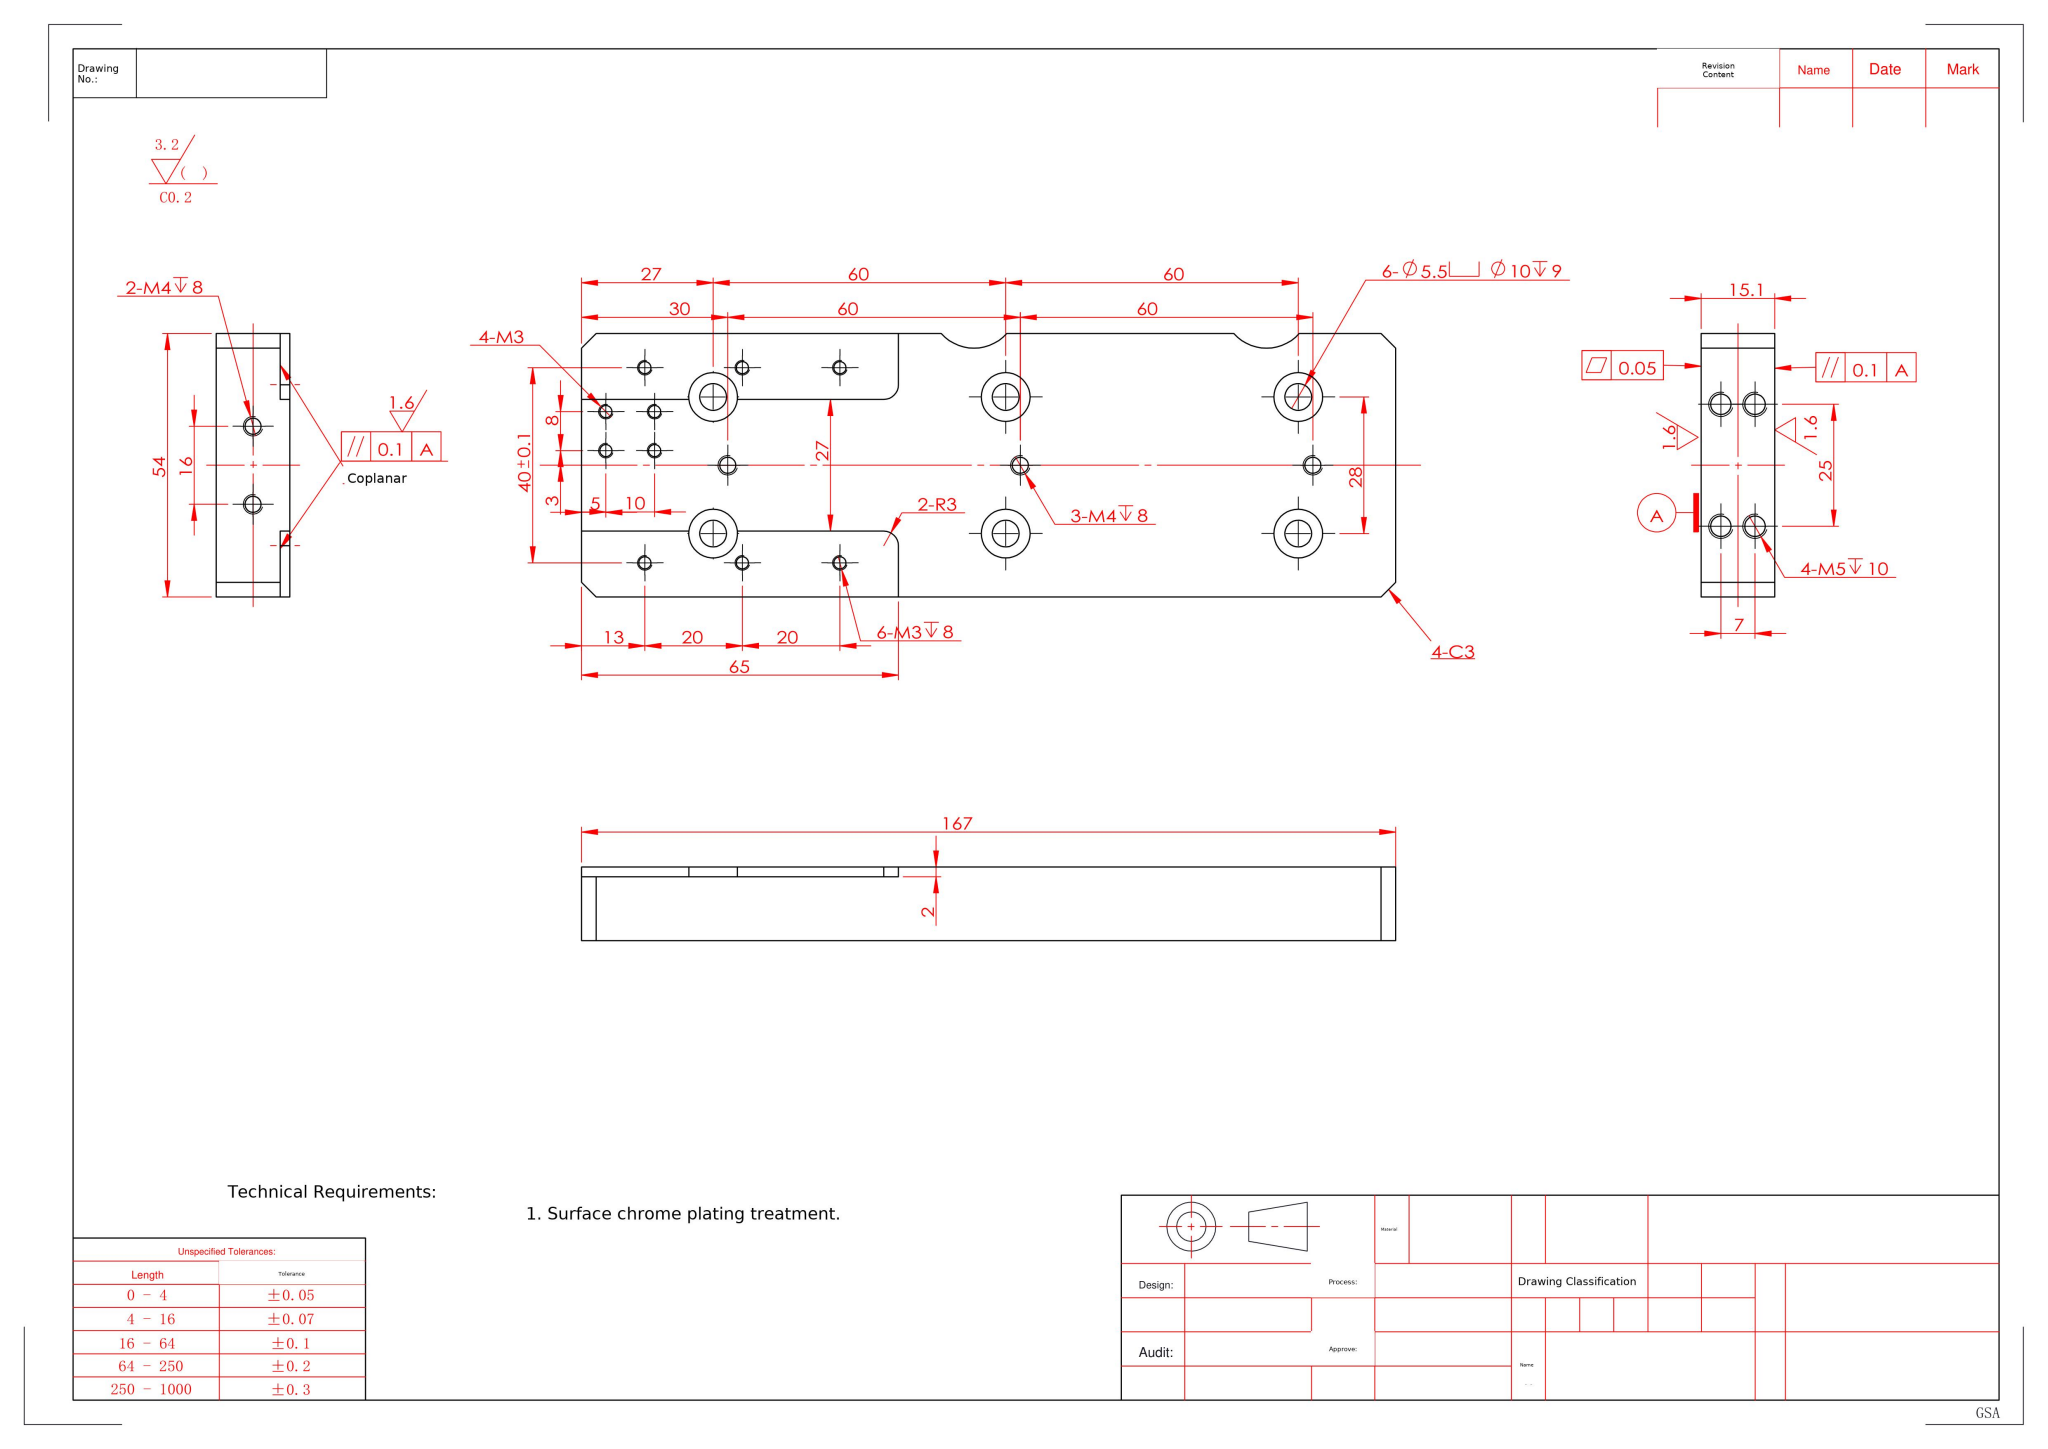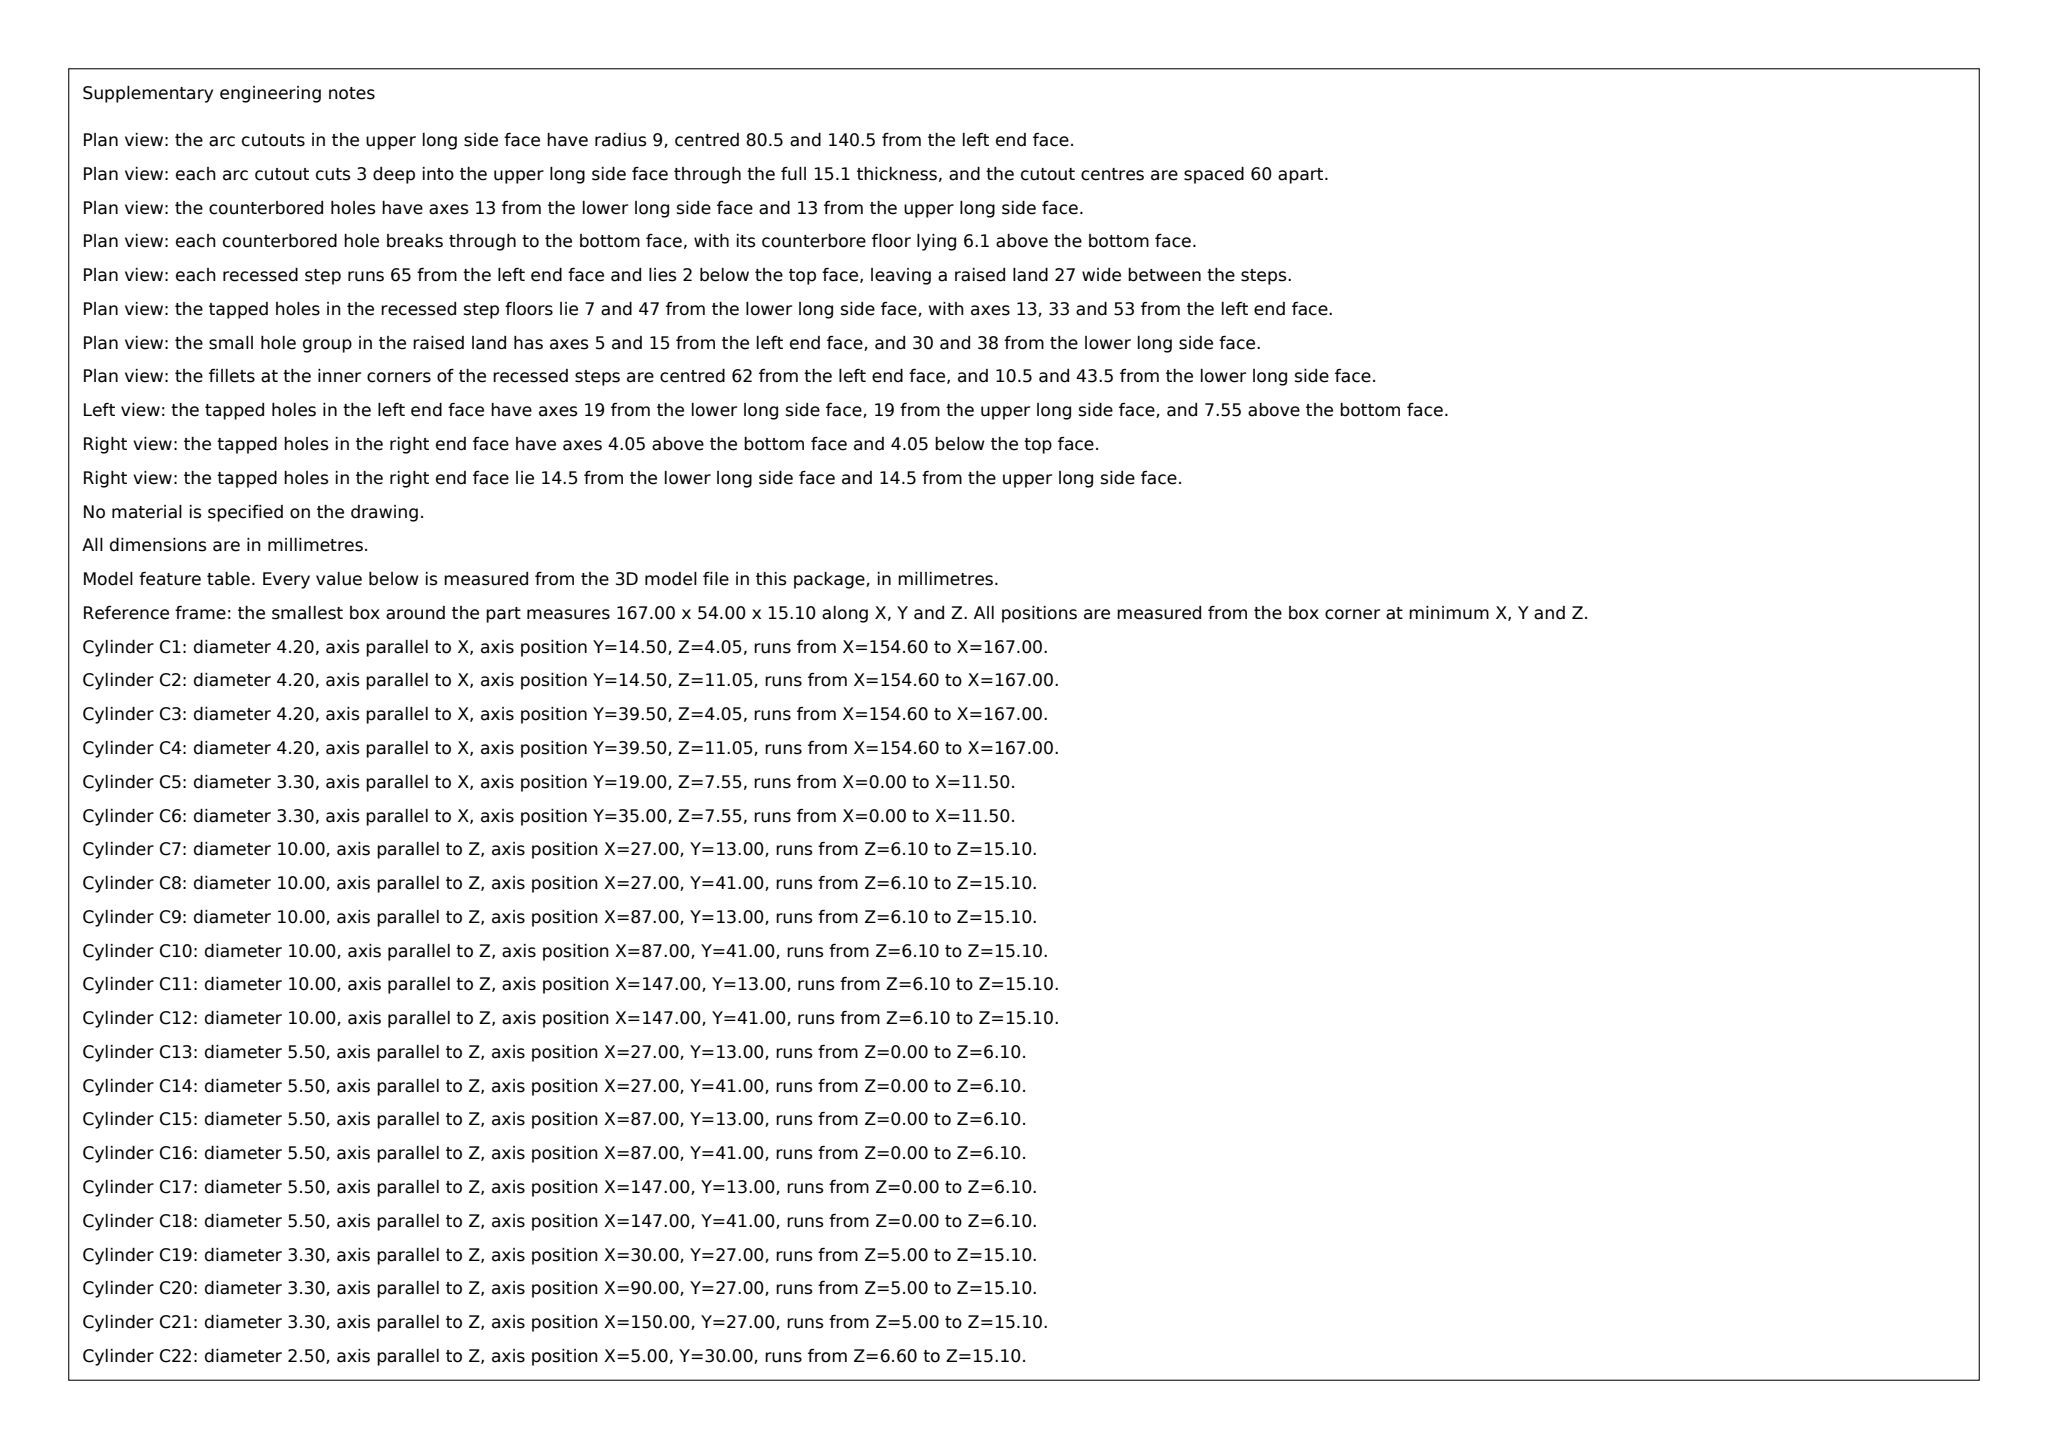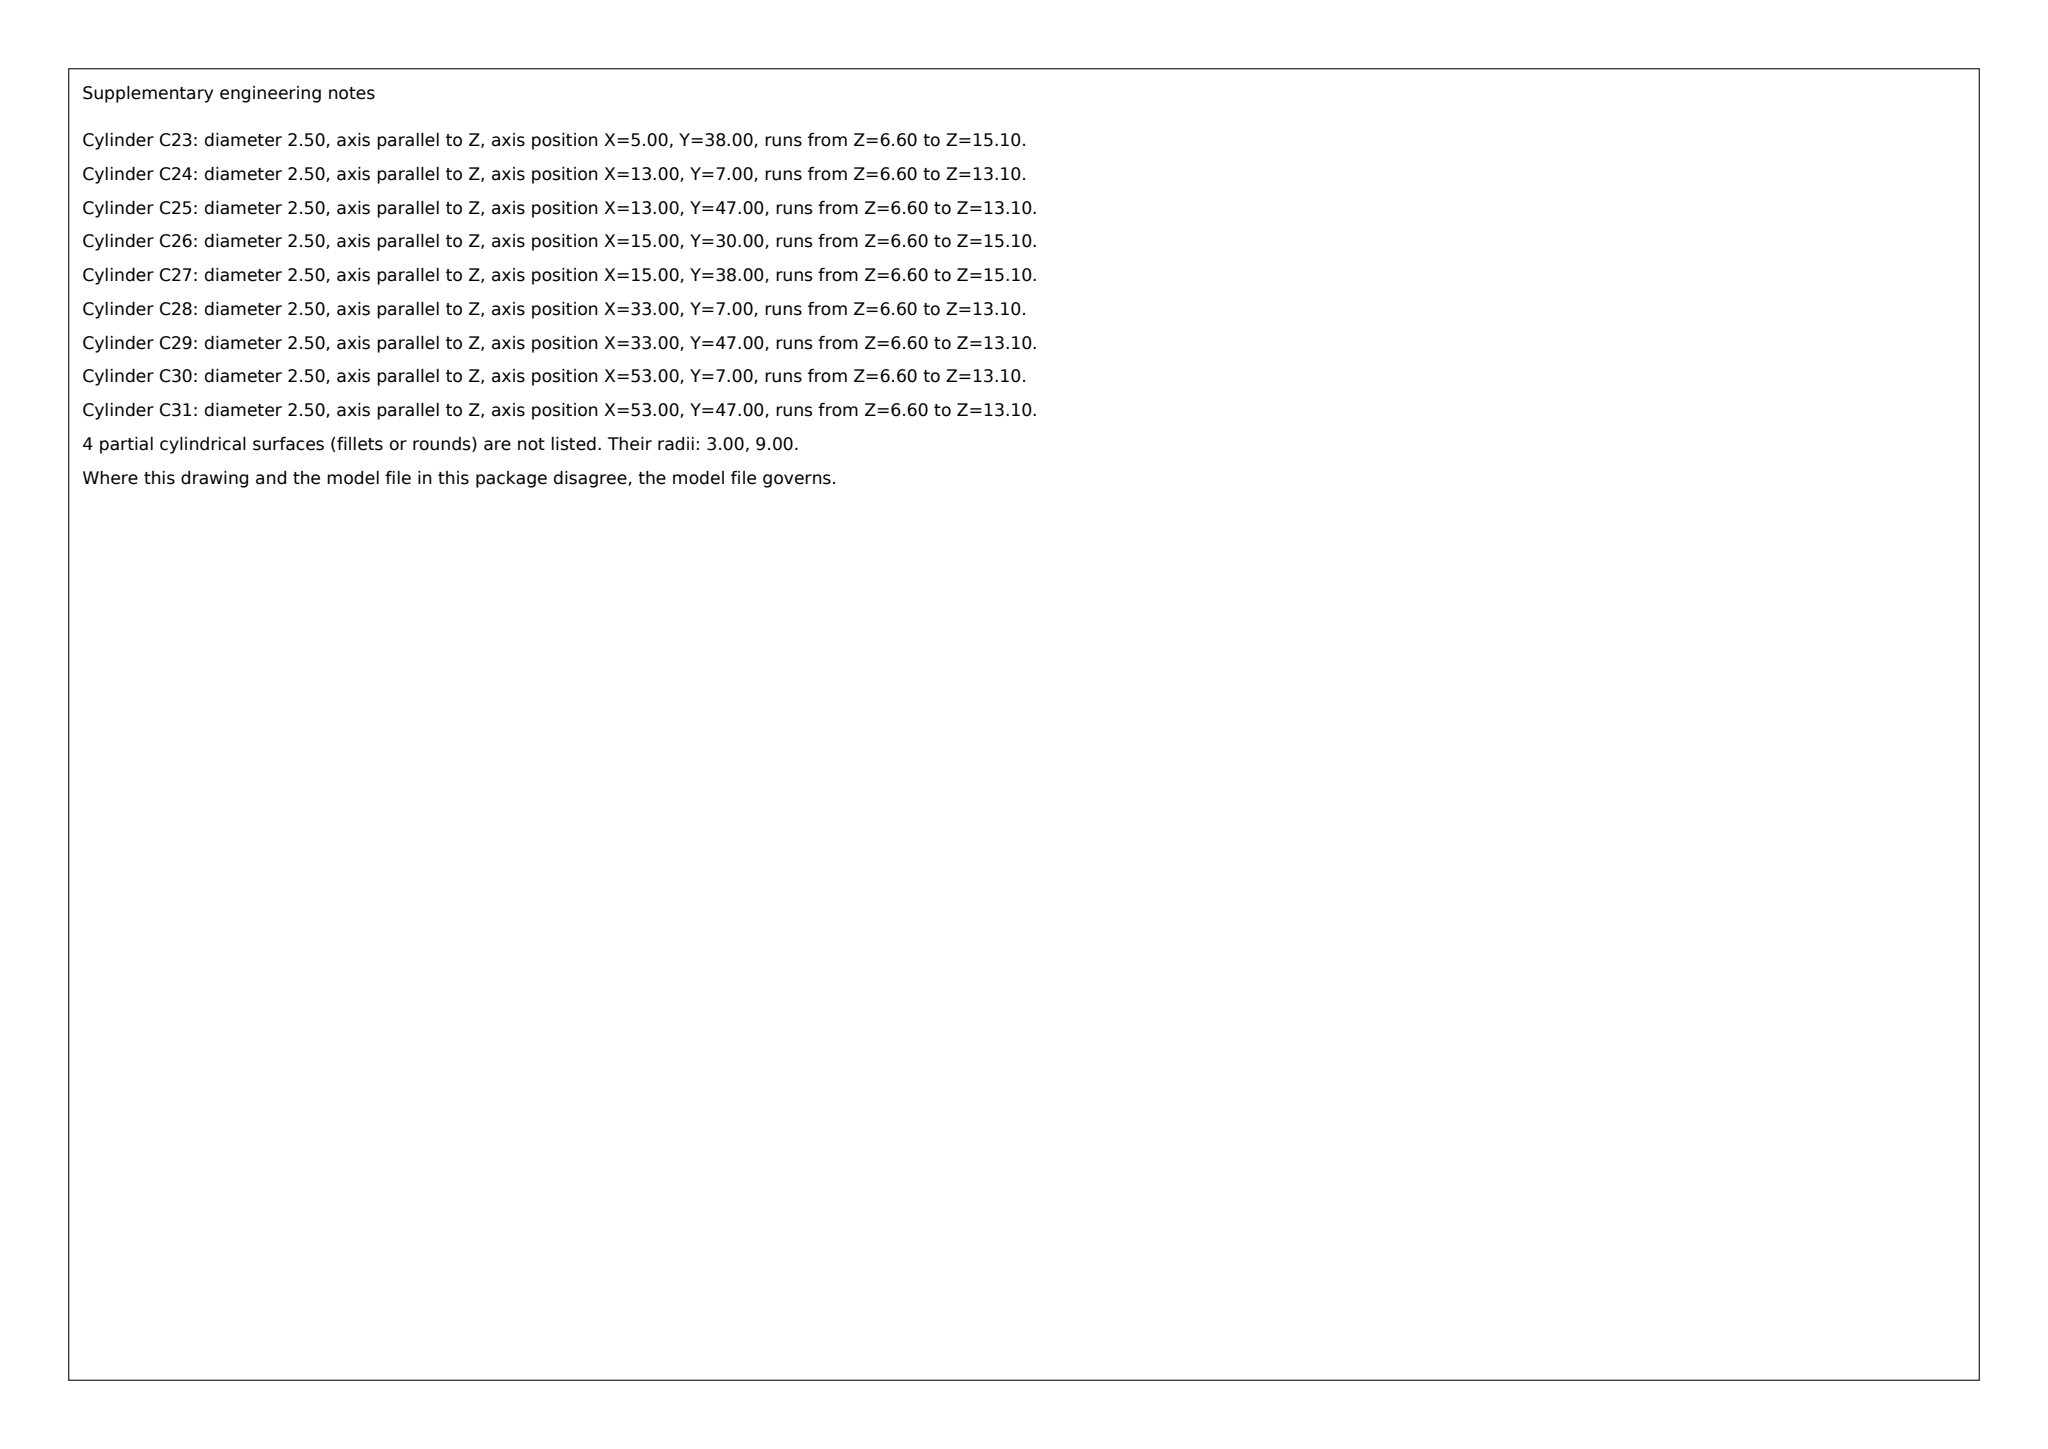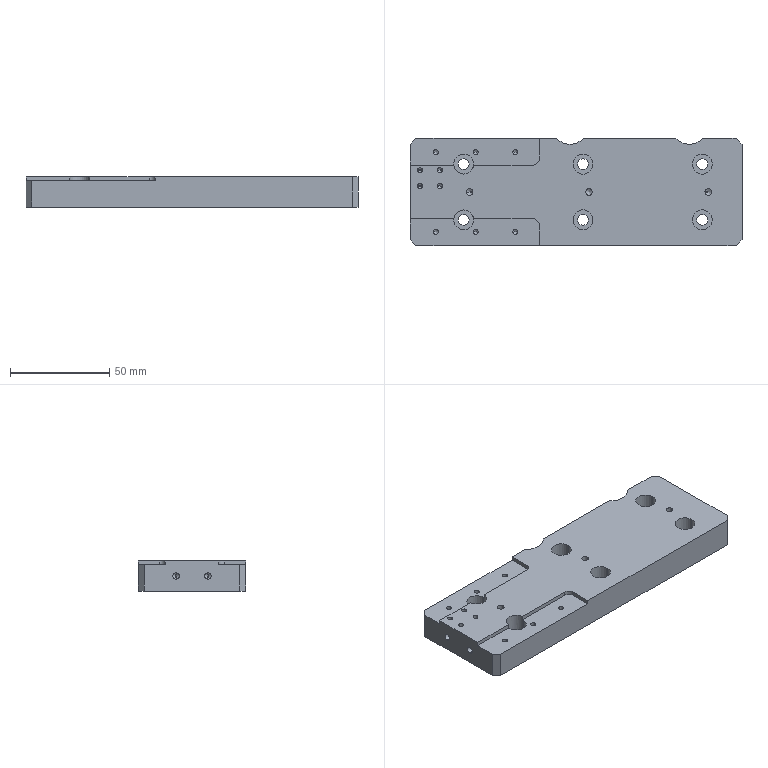Part | SolidWorks | mm | 1 solid | 130 faces | box 167 x 54 x 15.1 mm | volume 125089 mm3 | cylinder 66 | cone 38 | plane 26 | commonest cylinder face diameters 2.5 x20 10 x12 5.5 x12 3.3 x10 4.2 x8 6 x2 18 x2
Drawing notes:
TOP STEP DP 2: 13.5 WIDE EA SIDE OF CTR LAND, 27 BTWN WALLS, 65 LG | from the solid: z-planes 15.1 (top) & 13.1 (step floor) = 2 deep; y-planes 13.5 & 40.5 step walls; x-plane 65 step end; part width 54
2-R3 AT STEP WALL ENDS, X65, Y13.5 & Y40.5 FROM EDGE | from the solid: step walls y=13.5/40.5 meet end face x=65; 54 wide bbox
build123d program:
from build123d import *

# Parameters (mm, degrees)
SKETCH1_W                                       = 167
SKETCH1_H                                       = 54
BOSS_EXTRUDE1_DEPTH                             = 15.1
M5_HEX_SOCKET_HEAD_CAP_SCREW_CBORE1_D           = 5.5
M5_HEX_SOCKET_HEAD_CAP_SCREW_CBORE1_CBORE_D     = 10
M5_HEX_SOCKET_HEAD_CAP_SCREW_CBORE1_CBORE_DEPTH = 9
M4_TAPPED_HOLE1_D                               = 3.3
M4_TAPPED_HOLE1_DEPTH                           = 10.1
M4_TAPPED_HOLE1_TIP                             = 0.9914
CHAMFER1_SIZE                                   = 3
M5_TAPPED_HOLE1_D                               = 4.2
M5_TAPPED_HOLE1_DEPTH                           = 12.4
M5_TAPPED_HOLE1_TIP                             = 1.262
CUT_EXTRUDE1_DEPTH                              = 2
M3_TAPPED_HOLE1_D                               = 2.5
M3_TAPPED_HOLE1_DEPTH                           = 8.5
M3_TAPPED_HOLE1_TIP                             = 0.7511
M4_TAPPED_HOLE2_D                               = 3.3
M4_TAPPED_HOLE2_DEPTH                           = 11.5
M4_TAPPED_HOLE2_TIP                             = 0.9914
M3_TAPPED_HOLE2_D                               = 2.5
M3_TAPPED_HOLE2_DEPTH                           = 8.5
M3_TAPPED_HOLE2_TIP                             = 0.7511
SKETCH18_R                                      = 9
CUT_EXTRUDE4_DEPTH                              = 177.162


with BuildPart() as part:
    # Sketch1 → Boss-Extrude1 (new body)
    with BuildSketch(Plane.XY):
        with Locations((83.5, 27)):
            Rectangle(SKETCH1_W, SKETCH1_H)
    extrude(amount=BOSS_EXTRUDE1_DEPTH)

    # M5 Hex Socket Head Cap Screw CBORE1 (through all)
    with Locations(Plane.XY.offset(15.1)):
        with Locations((27, 41), (87, 41), (147, 41), (147, 13), (87, 13), (27, 13)):
            CounterBoreHole(M5_HEX_SOCKET_HEAD_CAP_SCREW_CBORE1_D / 2, M5_HEX_SOCKET_HEAD_CAP_SCREW_CBORE1_CBORE_D / 2, M5_HEX_SOCKET_HEAD_CAP_SCREW_CBORE1_CBORE_DEPTH)

    # M4 Tapped Hole1
    with Locations(Plane.XY.offset(15.1)):
        with Locations((30, 27), (90, 27), (150, 27)):
            Hole(M4_TAPPED_HOLE1_D / 2, depth=M4_TAPPED_HOLE1_DEPTH)
            with Locations((0, 0, -(M4_TAPPED_HOLE1_DEPTH + M4_TAPPED_HOLE1_TIP / 2))):  # 118° drill point
                Cone(0, M4_TAPPED_HOLE1_D / 2, M4_TAPPED_HOLE1_TIP, mode=Mode.SUBTRACT)

    # Chamfer1
    chamfer1_edges = [part.edges().sort_by_distance(p)[0] for p in [
        (0, 54, 7.55),
        (167, 54, 7.55),
        (167, 0, 7.55),
        (0, 0, 7.55),
    ]]
    chamfer(chamfer1_edges, length=CHAMFER1_SIZE)

    # M5 Tapped Hole1
    with Locations(Plane(origin=(167, 0, 0), x_dir=(0, 0, -1), z_dir=(1, 0, 0))):
        with Locations((-11.05, 14.5), (-4.05, 14.5), (-4.05, 39.5), (-11.05, 39.5)):
            Hole(M5_TAPPED_HOLE1_D / 2, depth=M5_TAPPED_HOLE1_DEPTH)
            with Locations((0, 0, -(M5_TAPPED_HOLE1_DEPTH + M5_TAPPED_HOLE1_TIP / 2))):  # 118° drill point
                Cone(0, M5_TAPPED_HOLE1_D / 2, M5_TAPPED_HOLE1_TIP, mode=Mode.SUBTRACT)

    # Sketch14 → Cut-Extrude1 (cut)
    with BuildSketch(Plane.XY.offset(15.1)):
        with BuildLine():
            Line((0, 40.5), (62, 40.5))
            ThreePointArc((62, 40.5), (64.121, 41.379), (65, 43.5))
            Line((65, 43.5), (65, 54))
            Line((65, 54), (0, 54))
            Line((0, 54), (0, 40.5))
        make_face()
        with BuildLine():
            Line((65, 10.5), (65, 0))
            Line((65, 0), (0, 0))
            Line((0, 0), (0, 13.5))
            Line((0, 13.5), (62, 13.5))
            ThreePointArc((62, 13.5), (64.121, 12.621), (65, 10.5))
        make_face()
    extrude(amount=-CUT_EXTRUDE1_DEPTH, mode=Mode.SUBTRACT)

    # M3 Tapped Hole1
    with Locations(Plane.XY.offset(15.1)):
        with Locations((13, 7), (33, 7), (53, 7), (13, 47), (33, 47), (53, 47)):
            Hole(M3_TAPPED_HOLE1_D / 2, depth=M3_TAPPED_HOLE1_DEPTH)
            with Locations((0, 0, -(M3_TAPPED_HOLE1_DEPTH + M3_TAPPED_HOLE1_TIP / 2))):  # 118° drill point
                Cone(0, M3_TAPPED_HOLE1_D / 2, M3_TAPPED_HOLE1_TIP, mode=Mode.SUBTRACT)

    # M4 Tapped Hole2
    with Locations(Plane.ZY):
        with Locations((7.55, 35), (7.55, 19)):
            Hole(M4_TAPPED_HOLE2_D / 2, depth=M4_TAPPED_HOLE2_DEPTH)
            with Locations((0, 0, -(M4_TAPPED_HOLE2_DEPTH + M4_TAPPED_HOLE2_TIP / 2))):  # 118° drill point
                Cone(0, M4_TAPPED_HOLE2_D / 2, M4_TAPPED_HOLE2_TIP, mode=Mode.SUBTRACT)

    # M3 Tapped Hole2
    with Locations(Plane.XY.offset(15.1)):
        with Locations((15, 38), (5, 38), (15, 30), (5, 30)):
            Hole(M3_TAPPED_HOLE2_D / 2, depth=M3_TAPPED_HOLE2_DEPTH)
            with Locations((0, 0, -(M3_TAPPED_HOLE2_DEPTH + M3_TAPPED_HOLE2_TIP / 2))):  # 118° drill point
                Cone(0, M3_TAPPED_HOLE2_D / 2, M3_TAPPED_HOLE2_TIP, mode=Mode.SUBTRACT)

    # Sketch18 → Cut-Extrude4 (cut, through all)
    with BuildSketch(Plane.XY):
        with Locations((140.5, 60)):
            Circle(SKETCH18_R)
        with Locations((80.5, 60)):
            Circle(SKETCH18_R)
    extrude(amount=CUT_EXTRUDE4_DEPTH, mode=Mode.SUBTRACT)


solid = part.part